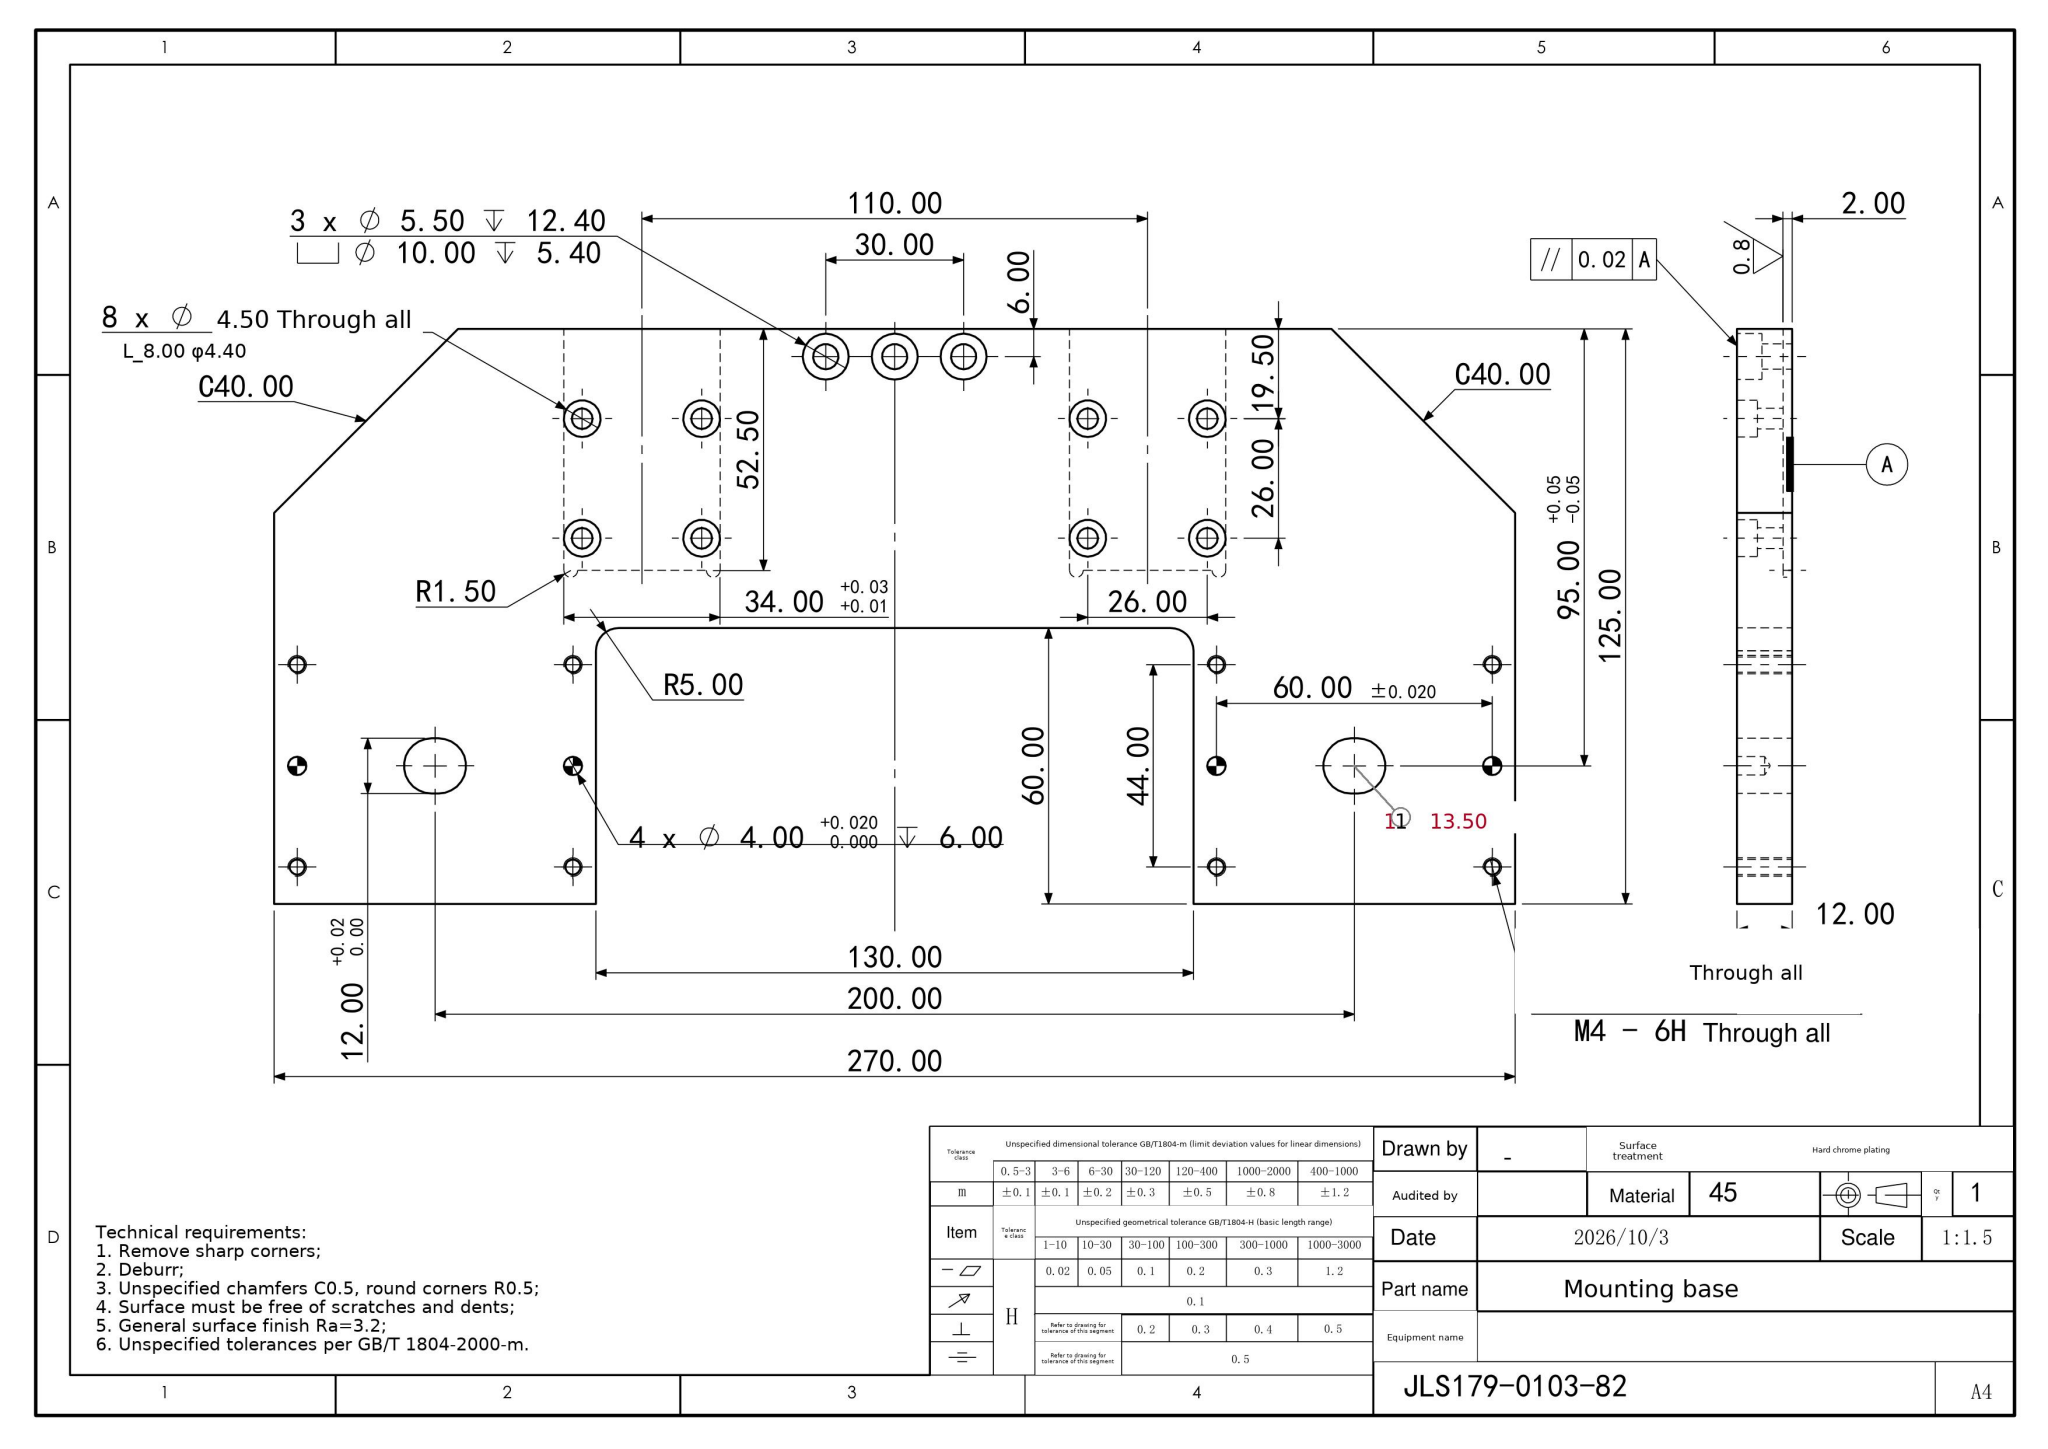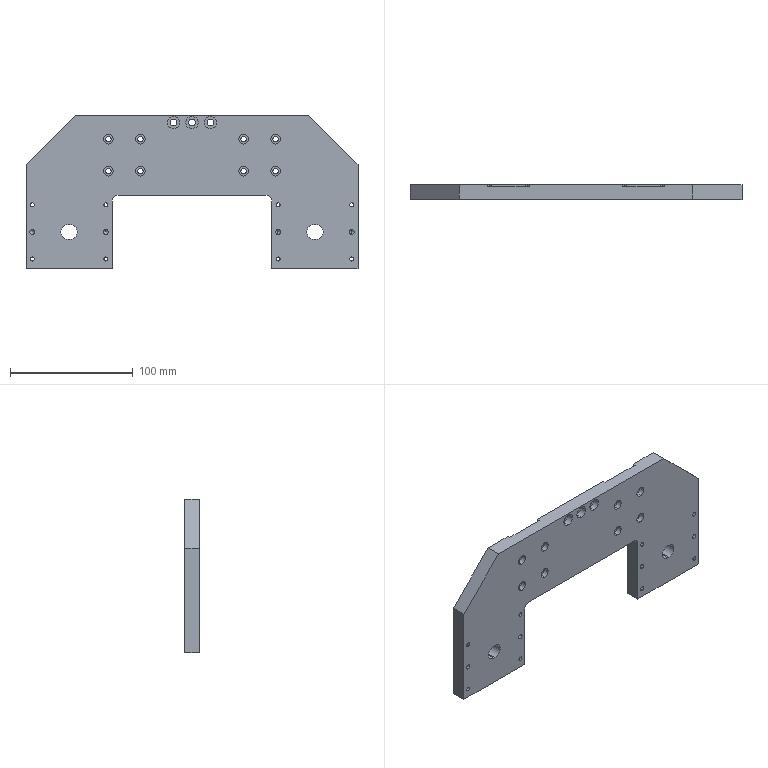Part | SolidWorks | mm | material 45 | 1 solid | 125 faces | box 270 x 12 x 125 mm | volume 276647 mm3 | cylinder 82 | plane 35 | cone 8 | commonest cylinder face diameters 8 x16 4.5 x16 3.3 x16 10 x8 4 x8 3 x8 5.5 x6 12 x4
build123d program:
from build123d import *

# Parameters (mm, degrees)
SKETCH1_W                                       = 270
SKETCH1_H                                       = 12
BOSS_EXTRUDE1_DEPTH                             = 65
SKETCH2_W                                       = 34
SKETCH2_H                                       = 130
CUT_EXTRUDE1_DEPTH                              = 2
SKETCH3_W                                       = 70
SKETCH3_H                                       = 12
BOSS_EXTRUDE2_DEPTH                             = 60
SKETCH4_W                                       = 34
SKETCH4_H                                       = 12.5
BOSS_EXTRUDE3_DEPTH                             = 2
SKETCH5_R                                       = 1.5
CUT_EXTRUDE2_DEPTH                              = 151.167
M4_TAPPED_HOLE1_D                               = 3.3
F_4_0MM_DOWEL_HOLE1_D                           = 4
F_4_0MM_DOWEL_HOLE1_DEPTH                       = 6
F_4_0MM_DOWEL_HOLE1_TIP                         = 1.202
FILLET1_R                                       = 5
M4_HEX_SOCKET_HEAD_CAP_SCREW_CBORE1_D           = 4.5
M4_HEX_SOCKET_HEAD_CAP_SCREW_CBORE1_CBORE_D     = 8
M4_HEX_SOCKET_HEAD_CAP_SCREW_CBORE1_CBORE_DEPTH = 4.4
CUT_EXTRUDE3_DEPTH                              = 151.313
M5_HEX_SOCKET_HEAD_CAP_SCREW_CBORE1_D           = 5.5
M5_HEX_SOCKET_HEAD_CAP_SCREW_CBORE1_DEPTH       = 12.4
M5_HEX_SOCKET_HEAD_CAP_SCREW_CBORE1_CBORE_D     = 10
M5_HEX_SOCKET_HEAD_CAP_SCREW_CBORE1_CBORE_DEPTH = 5.4
M5_HEX_SOCKET_HEAD_CAP_SCREW_CBORE1_TIP         = 1.652
SKETCH15_R                                      = 6
SKETCH15_R_2                                    = 6
CUT_EXTRUDE4_DEPTH                              = 151.313
CUT_EXTRUDE5_DEPTH                              = 151.313


with BuildPart() as part:
    # Sketch1 → Boss-Extrude1 (new body)
    with BuildSketch(Plane.XY):
        Rectangle(SKETCH1_W, SKETCH1_H)
    extrude(amount=BOSS_EXTRUDE1_DEPTH)

    # Sketch2 → Cut-Extrude1 (cut)
    with BuildSketch(Plane(origin=(0, 6, 0), x_dir=(1, 0, 0), z_dir=(0, 1, 0))):
        with Locations((55, 0)):
            Rectangle(SKETCH2_W, SKETCH2_H)
        with Locations((-55, 0)):
            Rectangle(SKETCH2_W, SKETCH2_H)
    extrude(amount=-CUT_EXTRUDE1_DEPTH, mode=Mode.SUBTRACT)

    # Sketch3 → Boss-Extrude2 (add)
    with BuildSketch(Plane(origin=(0, 0, 0), x_dir=(-1, 0, 0), z_dir=(0, 0, -1))):
        with Locations((100, 0)):
            Rectangle(SKETCH3_W, SKETCH3_H)
        with Locations((-100, 0)):
            Rectangle(SKETCH3_W, SKETCH3_H)
    extrude(amount=BOSS_EXTRUDE2_DEPTH)

    # Sketch4 → Boss-Extrude3 (add)
    with BuildSketch(Plane(origin=(0, 4, 0), x_dir=(1, 0, 0), z_dir=(0, 1, 0))):
        with Locations((55, -6.25)):
            Rectangle(SKETCH4_W, SKETCH4_H)
        with Locations((-55, -6.25)):
            Rectangle(SKETCH4_W, SKETCH4_H)
    extrude(amount=BOSS_EXTRUDE3_DEPTH)

    # Sketch5 → Cut-Extrude2 (cut, through all)
    with BuildSketch(Plane(origin=(0, 4, 0), x_dir=(1, 0, 0), z_dir=(0, 1, 0))):
        with Locations((39.5, -12.5)):
            Circle(SKETCH5_R)
        with Locations((70.5, -12.5)):
            Circle(SKETCH5_R)
        with Locations((-70.5, -12.5)):
            Circle(SKETCH5_R)
        with Locations((-39.5, -12.5)):
            Circle(SKETCH5_R)
    extrude(amount=CUT_EXTRUDE2_DEPTH, mode=Mode.SUBTRACT)

    # M4 Tapped Hole1 (through all)
    with Locations(Plane(origin=(0, -6, 0), x_dir=(-1, 0, 0), z_dir=(0, -1, 0))):
        with Locations((130, 52), (130, 8), (70, 8), (70, 52), (-70, 52), (-70, 8), (-130, 8), (-130, 52)):
            Hole(M4_TAPPED_HOLE1_D / 2)

    # 4.0mm Dowel Hole1
    with Locations(Plane(origin=(0, -6, 0), x_dir=(-1, 0, 0), z_dir=(0, -1, 0))):
        with Locations((-70, 30), (-130, 30), (130, 30), (70, 30)):
            Hole(F_4_0MM_DOWEL_HOLE1_D / 2, depth=F_4_0MM_DOWEL_HOLE1_DEPTH)
            with Locations((0, 0, -(F_4_0MM_DOWEL_HOLE1_DEPTH + F_4_0MM_DOWEL_HOLE1_TIP / 2))):  # 118° drill point
                Cone(0, F_4_0MM_DOWEL_HOLE1_D / 2, F_4_0MM_DOWEL_HOLE1_TIP, mode=Mode.SUBTRACT)

    # Fillet1
    fillet1_edges = [part.edges().sort_by_distance(p)[0] for p in [
        (-65, 0, 0),
        (65, 0, 0),
    ]]
    fillet(fillet1_edges, radius=FILLET1_R)

    # M4 Hex Socket Head Cap Screw CBORE1 (through all)
    with Locations(Plane(origin=(0, -6, 0), x_dir=(-1, 0, 0), z_dir=(0, -1, 0))):
        with Locations((-42, -19.5), (-68, -19.5), (-42, -45.5), (-68, -45.5), (42, -19.5), (68, -19.5), (68, -45.5), (42, -45.5)):
            CounterBoreHole(M4_HEX_SOCKET_HEAD_CAP_SCREW_CBORE1_D / 2, M4_HEX_SOCKET_HEAD_CAP_SCREW_CBORE1_CBORE_D / 2, M4_HEX_SOCKET_HEAD_CAP_SCREW_CBORE1_CBORE_DEPTH)

    # Sketch12 → Cut-Extrude3 (cut, through all)
    with BuildSketch(Plane(origin=(0, -6, 0), x_dir=(-1, 0, 0), z_dir=(0, -1, 0))):
        Polygon((-135, -25), (-95, -65), (-135, -65), align=None)
        Polygon((135, -65), (135, -25), (95, -65), align=None)
    extrude(amount=-CUT_EXTRUDE3_DEPTH, mode=Mode.SUBTRACT)

    # M5 Hex Socket Head Cap Screw CBORE1
    with Locations(Plane(origin=(0, -6, 0), x_dir=(-1, 0, 0), z_dir=(0, -1, 0))):
        with Locations((15, -59), (0, -59), (-15, -59)):
            CounterBoreHole(M5_HEX_SOCKET_HEAD_CAP_SCREW_CBORE1_D / 2, M5_HEX_SOCKET_HEAD_CAP_SCREW_CBORE1_CBORE_D / 2, M5_HEX_SOCKET_HEAD_CAP_SCREW_CBORE1_CBORE_DEPTH, depth=M5_HEX_SOCKET_HEAD_CAP_SCREW_CBORE1_DEPTH)
            with Locations((0, 0, -(M5_HEX_SOCKET_HEAD_CAP_SCREW_CBORE1_DEPTH + M5_HEX_SOCKET_HEAD_CAP_SCREW_CBORE1_TIP / 2))):  # 118° drill point
                Cone(0, M5_HEX_SOCKET_HEAD_CAP_SCREW_CBORE1_D / 2, M5_HEX_SOCKET_HEAD_CAP_SCREW_CBORE1_TIP, mode=Mode.SUBTRACT)

    # Sketch15 → Cut-Extrude4 (cut, through all)
    with BuildSketch(Plane(origin=(0, -6, 0), x_dir=(-1, 0, 0), z_dir=(0, -1, 0))):
        with Locations(Location((-100, 30, 0), (0, 0, 90))):
            Circle(SKETCH15_R)
        with Locations(Location((100, 30, 0), (0, 0, 90))):
            Circle(SKETCH15_R_2)
    extrude(amount=-CUT_EXTRUDE4_DEPTH, mode=Mode.SUBTRACT)

    # Sketch16 → Cut-Extrude5 (cut, through all)
    with BuildSketch(Plane(origin=(0, -6, 0), x_dir=(-1, 0, 0), z_dir=(0, -1, 0))):
        with BuildLine():
            Line((-99.25, 24), (-100.75, 24))
            ThreePointArc((-100.75, 24), (-106.75, 30), (-100.75, 36))
            Line((-100.75, 36), (-99.25, 36))
            ThreePointArc((-99.25, 36), (-93.25, 30), (-99.25, 24))
        make_face()
        with BuildLine():
            Line((99.25, 24), (100.75, 24))
            ThreePointArc((100.75, 24), (106.75, 30), (100.75, 36))
            Line((100.75, 36), (99.25, 36))
            ThreePointArc((99.25, 36), (93.25, 30), (99.25, 24))
        make_face()
    extrude(amount=-CUT_EXTRUDE5_DEPTH, mode=Mode.SUBTRACT)


solid = part.part